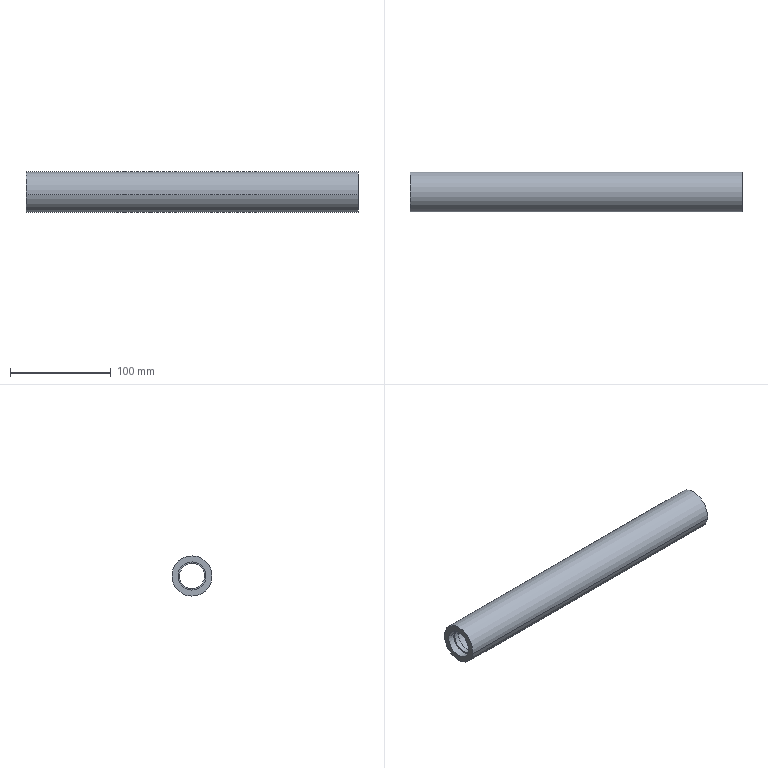Component | SolidWorks | 01-13MarkingMachinePrintingRoller-1 | 1 solid | 18 faces | box 330 x 40 x 40 mm | volume 123337 mm3 | cylinder 12 | plane 6 | commonest cylinder face diameters 28 x4 25 x4 40 x2 34 x2 | material A3 Steel
build123d program:
from build123d import *


with BuildPart() as part:
    # Sketch1 → Revolve1 (revolve)
    with BuildSketch(Plane.XY, mode=Mode.PRIVATE) as revolve1_sk:
        Polygon((-165, 20), (165, 20), (165, 14), (158, 14), (158, 12.5), (153, 12.5), (153, 17), (-153, 17), (-153, 12.5), (-158, 12.5), (-158, 14), (-165, 14), align=None)
    revolve(revolve1_sk.sketch.rotate(Axis((-220.554, 0, 0), (1, 0, 0)), 90), axis=Axis((-220.554, 0, 0), (1, 0, 0)))


solid = part.part

# Placed as in the assembly
solid = solid.moved(Location((-256.91, 2.41, 6.568), (0, 0, 0)))
STEP:
#1=COLOUR_RGB('',0.7922,0.8196,0.9333);
#2=FILL_AREA_STYLE_COLOUR('',#1);
#3=FILL_AREA_STYLE('',(#2));
#4=SURFACE_STYLE_FILL_AREA(#3);
#5=SURFACE_SIDE_STYLE('',(#4));
#6=SURFACE_STYLE_USAGE(.BOTH.,#5);
#7=PRESENTATION_STYLE_ASSIGNMENT((#6));
#8=CARTESIAN_POINT('',(-3.619,0.8756,0.3613));
#9=VERTEX_POINT('',#8);
#10=CARTESIAN_POINT('',(-3.619,-0.6858,0.1558));
#11=VERTEX_POINT('',#10);
#12=CARTESIAN_POINT('',(-3.619,0.0949,0.2586));
#13=DIRECTION('',(-1.,0.,0.));
#14=DIRECTION('',(0.,0.9915,0.1305));
#15=AXIS2_PLACEMENT_3D('',#12,#13,#14);
#16=CIRCLE('',#15,0.7874);
#17=EDGE_CURVE('',#9,#11,#16,.T.);
#18=ORIENTED_EDGE('',*,*,#17,.T.);
#19=CARTESIAN_POINT('',(-16.611,-0.6858,0.1558));
#20=VERTEX_POINT('',#19);
#21=CARTESIAN_POINT('',(-18.798,-0.6858,0.1558));
#22=DIRECTION('',(-1.,0.,0.));
#23=VECTOR('',#22,39.37);
#24=LINE('',#21,#23);
#25=EDGE_CURVE('',#11,#20,#24,.T.);
#26=ORIENTED_EDGE('',*,*,#25,.T.);
#27=CARTESIAN_POINT('',(-16.611,0.8756,0.3613));
#28=VERTEX_POINT('',#27);
#29=CARTESIAN_POINT('',(-16.611,0.0949,0.2586));
#30=DIRECTION('',(-1.,0.,0.));
#31=DIRECTION('',(0.,0.9915,0.1305));
#32=AXIS2_PLACEMENT_3D('',#29,#30,#31);
#33=CIRCLE('',#32,0.7874);
#34=EDGE_CURVE('',#28,#20,#33,.T.);
#35=ORIENTED_EDGE('',*,*,#34,.F.);
#36=CARTESIAN_POINT('',(-18.798,0.8756,0.3613));
#37=DIRECTION('',(-1.,0.,0.));
#38=VECTOR('',#37,39.37);
#39=LINE('',#36,#38);
#40=EDGE_CURVE('',#9,#28,#39,.T.);
#41=ORIENTED_EDGE('',*,*,#40,.F.);
#42=EDGE_LOOP('',(#18,#26,#35,#41));
#43=FACE_OUTER_BOUND('',#42,.T.);
#44=CARTESIAN_POINT('',(-18.798,0.0949,0.2586));
#45=DIRECTION('',(-1.,0.,0.));
#46=DIRECTION('',(0.,0.9915,0.1305));
#47=AXIS2_PLACEMENT_3D('',#44,#45,#46);
#48=CYLINDRICAL_SURFACE('',#47,0.7874);
#49=ADVANCED_FACE('',(#43),#48,.T.);
#50=CARTESIAN_POINT('',(-3.619,-0.4516,0.1867));
#51=VERTEX_POINT('',#50);
#52=CARTESIAN_POINT('',(-3.619,0.6414,0.3305));
#53=VERTEX_POINT('',#52);
#54=CARTESIAN_POINT('',(-3.619,0.0949,0.2586));
#55=DIRECTION('',(-1.,0.,0.));
#56=DIRECTION('',(0.,0.9915,0.1305));
#57=AXIS2_PLACEMENT_3D('',#54,#55,#56);
#58=CIRCLE('',#57,0.5512);
#59=EDGE_CURVE('',#51,#53,#58,.T.);
#60=ORIENTED_EDGE('',*,*,#59,.F.);
#61=CARTESIAN_POINT('',(-3.894,-0.4516,0.1867));
#62=VERTEX_POINT('',#61);
#63=CARTESIAN_POINT('',(-18.798,-0.4516,0.1867));
#64=DIRECTION('',(-1.,0.,0.));
#65=VECTOR('',#64,39.37);
#66=LINE('',#63,#65);
#67=EDGE_CURVE('',#51,#62,#66,.T.);
#68=ORIENTED_EDGE('',*,*,#67,.T.);
#69=CARTESIAN_POINT('',(-3.894,0.6414,0.3305));
#70=VERTEX_POINT('',#69);
#71=CARTESIAN_POINT('',(-3.894,0.0949,0.2586));
#72=DIRECTION('',(-1.,0.,0.));
#73=DIRECTION('',(0.,0.9915,0.1305));
#74=AXIS2_PLACEMENT_3D('',#71,#72,#73);
#75=CIRCLE('',#74,0.5512);
#76=EDGE_CURVE('',#62,#70,#75,.T.);
#77=ORIENTED_EDGE('',*,*,#76,.T.);
#78=CARTESIAN_POINT('',(-18.798,0.6414,0.3305));
#79=DIRECTION('',(-1.,0.,0.));
#80=VECTOR('',#79,39.37);
#81=LINE('',#78,#80);
#82=EDGE_CURVE('',#53,#70,#81,.T.);
#83=ORIENTED_EDGE('',*,*,#82,.F.);
#84=EDGE_LOOP('',(#60,#68,#77,#83));
#85=FACE_OUTER_BOUND('',#84,.T.);
#86=CARTESIAN_POINT('',(-18.798,0.0949,0.2586));
#87=DIRECTION('',(-1.,0.,0.));
#88=DIRECTION('',(0.,0.9915,0.1305));
#89=AXIS2_PLACEMENT_3D('',#86,#87,#88);
#90=CYLINDRICAL_SURFACE('',#89,0.5512);
#91=ADVANCED_FACE('',(#85),#90,.F.);
#92=CARTESIAN_POINT('',(-3.894,-0.393,0.1944));
#93=VERTEX_POINT('',#92);
#94=CARTESIAN_POINT('',(-3.894,0.5828,0.3228));
#95=VERTEX_POINT('',#94);
#96=CARTESIAN_POINT('',(-3.894,0.0949,0.2586));
#97=DIRECTION('',(-1.,0.,0.));
#98=DIRECTION('',(0.,0.9915,0.1305));
#99=AXIS2_PLACEMENT_3D('',#96,#97,#98);
#100=CIRCLE('',#99,0.4921);
#101=EDGE_CURVE('',#93,#95,#100,.T.);
#102=ORIENTED_EDGE('',*,*,#101,.F.);
#103=CARTESIAN_POINT('',(-4.091,-0.393,0.1944));
#104=VERTEX_POINT('',#103);
#105=CARTESIAN_POINT('',(-18.798,-0.393,0.1944));
#106=DIRECTION('',(-1.,0.,0.));
#107=VECTOR('',#106,39.37);
#108=LINE('',#105,#107);
#109=EDGE_CURVE('',#93,#104,#108,.T.);
#110=ORIENTED_EDGE('',*,*,#109,.T.);
#111=CARTESIAN_POINT('',(-4.091,0.5828,0.3228));
#112=VERTEX_POINT('',#111);
#113=CARTESIAN_POINT('',(-4.091,0.0949,0.2586));
#114=DIRECTION('',(-1.,0.,0.));
#115=DIRECTION('',(0.,0.9915,0.1305));
#116=AXIS2_PLACEMENT_3D('',#113,#114,#115);
#117=CIRCLE('',#116,0.4921);
#118=EDGE_CURVE('',#104,#112,#117,.T.);
#119=ORIENTED_EDGE('',*,*,#118,.T.);
#120=CARTESIAN_POINT('',(-18.798,0.5828,0.3228));
#121=DIRECTION('',(-1.,0.,0.));
#122=VECTOR('',#121,39.37);
#123=LINE('',#120,#122);
#124=EDGE_CURVE('',#95,#112,#123,.T.);
#125=ORIENTED_EDGE('',*,*,#124,.F.);
#126=EDGE_LOOP('',(#102,#110,#119,#125));
#127=FACE_OUTER_BOUND('',#126,.T.);
#128=CARTESIAN_POINT('',(-18.798,0.0949,0.2586));
#129=DIRECTION('',(-1.,0.,0.));
#130=DIRECTION('',(0.,0.9915,0.1305));
#131=AXIS2_PLACEMENT_3D('',#128,#129,#130);
#132=CYLINDRICAL_SURFACE('',#131,0.4921);
#133=ADVANCED_FACE('',(#127),#132,.F.);
#134=CARTESIAN_POINT('',(-4.091,-0.5687,0.1713));
#135=VERTEX_POINT('',#134);
#136=CARTESIAN_POINT('',(-4.091,0.7585,0.3459));
#137=VERTEX_POINT('',#136);
#138=CARTESIAN_POINT('',(-4.091,0.0949,0.2586));
#139=DIRECTION('',(-1.,0.,0.));
#140=DIRECTION('',(0.,0.9915,0.1305));
#141=AXIS2_PLACEMENT_3D('',#138,#139,#140);
#142=CIRCLE('',#141,0.6693);
#143=EDGE_CURVE('',#135,#137,#142,.T.);
#144=ORIENTED_EDGE('',*,*,#143,.F.);
#145=CARTESIAN_POINT('',(-16.138,-0.5687,0.1713));
#146=VERTEX_POINT('',#145);
#147=CARTESIAN_POINT('',(-18.798,-0.5687,0.1713));
#148=DIRECTION('',(-1.,0.,0.));
#149=VECTOR('',#148,39.37);
#150=LINE('',#147,#149);
#151=EDGE_CURVE('',#135,#146,#150,.T.);
#152=ORIENTED_EDGE('',*,*,#151,.T.);
#153=CARTESIAN_POINT('',(-16.138,0.7585,0.3459));
#154=VERTEX_POINT('',#153);
#155=CARTESIAN_POINT('',(-16.138,0.0949,0.2586));
#156=DIRECTION('',(-1.,0.,0.));
#157=DIRECTION('',(0.,0.9915,0.1305));
#158=AXIS2_PLACEMENT_3D('',#155,#156,#157);
#159=CIRCLE('',#158,0.6693);
#160=EDGE_CURVE('',#146,#154,#159,.T.);
#161=ORIENTED_EDGE('',*,*,#160,.T.);
#162=CARTESIAN_POINT('',(-18.798,0.7585,0.3459));
#163=DIRECTION('',(-1.,0.,0.));
#164=VECTOR('',#163,39.37);
#165=LINE('',#162,#164);
#166=EDGE_CURVE('',#137,#154,#165,.T.);
#167=ORIENTED_EDGE('',*,*,#166,.F.);
#168=EDGE_LOOP('',(#144,#152,#161,#167));
#169=FACE_OUTER_BOUND('',#168,.T.);
#170=CARTESIAN_POINT('',(-18.798,0.0949,0.2586));
#171=DIRECTION('',(-1.,0.,0.));
#172=DIRECTION('',(0.,0.9915,0.1305));
#173=AXIS2_PLACEMENT_3D('',#170,#171,#172);
#174=CYLINDRICAL_SURFACE('',#173,0.6693);
#175=ADVANCED_FACE('',(#169),#174,.F.);
#176=CARTESIAN_POINT('',(-16.138,-0.393,0.1944));
#177=VERTEX_POINT('',#176);
#178=CARTESIAN_POINT('',(-16.138,0.5828,0.3228));
#179=VERTEX_POINT('',#178);
#180=CARTESIAN_POINT('',(-16.138,0.0949,0.2586));
#181=DIRECTION('',(-1.,0.,0.));
#182=DIRECTION('',(0.,0.9915,0.1305));
#183=AXIS2_PLACEMENT_3D('',#180,#181,#182);
#184=CIRCLE('',#183,0.4921);
#185=EDGE_CURVE('',#177,#179,#184,.T.);
#186=ORIENTED_EDGE('',*,*,#185,.F.);
#187=CARTESIAN_POINT('',(-16.335,-0.393,0.1944));
#188=VERTEX_POINT('',#187);
#189=CARTESIAN_POINT('',(-18.798,-0.393,0.1944));
#190=DIRECTION('',(-1.,0.,0.));
#191=VECTOR('',#190,39.37);
#192=LINE('',#189,#191);
#193=EDGE_CURVE('',#177,#188,#192,.T.);
#194=ORIENTED_EDGE('',*,*,#193,.T.);
#195=CARTESIAN_POINT('',(-16.335,0.5828,0.3228));
#196=VERTEX_POINT('',#195);
#197=CARTESIAN_POINT('',(-16.335,0.0949,0.2586));
#198=DIRECTION('',(-1.,0.,0.));
#199=DIRECTION('',(0.,0.9915,0.1305));
#200=AXIS2_PLACEMENT_3D('',#197,#198,#199);
#201=CIRCLE('',#200,0.4921);
#202=EDGE_CURVE('',#188,#196,#201,.T.);
#203=ORIENTED_EDGE('',*,*,#202,.T.);
#204=CARTESIAN_POINT('',(-18.798,0.5828,0.3228));
#205=DIRECTION('',(-1.,0.,0.));
#206=VECTOR('',#205,39.37);
#207=LINE('',#204,#206);
#208=EDGE_CURVE('',#179,#196,#207,.T.);
#209=ORIENTED_EDGE('',*,*,#208,.F.);
#210=EDGE_LOOP('',(#186,#194,#203,#209));
#211=FACE_OUTER_BOUND('',#210,.T.);
#212=CARTESIAN_POINT('',(-18.798,0.0949,0.2586));
#213=DIRECTION('',(-1.,0.,0.));
#214=DIRECTION('',(0.,0.9915,0.1305));
#215=AXIS2_PLACEMENT_3D('',#212,#213,#214);
#216=CYLINDRICAL_SURFACE('',#215,0.4921);
#217=ADVANCED_FACE('',(#211),#216,.F.);
#218=CARTESIAN_POINT('',(-16.335,-0.4516,0.1867));
#219=VERTEX_POINT('',#218);
#220=CARTESIAN_POINT('',(-16.335,0.6414,0.3305));
#221=VERTEX_POINT('',#220);
#222=CARTESIAN_POINT('',(-16.335,0.0949,0.2586));
#223=DIRECTION('',(-1.,0.,0.));
#224=DIRECTION('',(0.,0.9915,0.1305));
#225=AXIS2_PLACEMENT_3D('',#222,#223,#224);
#226=CIRCLE('',#225,0.5512);
#227=EDGE_CURVE('',#219,#221,#226,.T.);
#228=ORIENTED_EDGE('',*,*,#227,.F.);
#229=CARTESIAN_POINT('',(-16.611,-0.4516,0.1867));
#230=VERTEX_POINT('',#229);
#231=CARTESIAN_POINT('',(-18.798,-0.4516,0.1867));
#232=DIRECTION('',(-1.,0.,0.));
#233=VECTOR('',#232,39.37);
#234=LINE('',#231,#233);
#235=EDGE_CURVE('',#219,#230,#234,.T.);
#236=ORIENTED_EDGE('',*,*,#235,.T.);
#237=CARTESIAN_POINT('',(-16.611,0.6414,0.3305));
#238=VERTEX_POINT('',#237);
#239=CARTESIAN_POINT('',(-16.611,0.0949,0.2586));
#240=DIRECTION('',(-1.,0.,0.));
#241=DIRECTION('',(0.,0.9915,0.1305));
#242=AXIS2_PLACEMENT_3D('',#239,#240,#241);
#243=CIRCLE('',#242,0.5512);
#244=EDGE_CURVE('',#230,#238,#243,.T.);
#245=ORIENTED_EDGE('',*,*,#244,.T.);
#246=CARTESIAN_POINT('',(-18.798,0.6414,0.3305));
#247=DIRECTION('',(-1.,0.,0.));
#248=VECTOR('',#247,39.37);
#249=LINE('',#246,#248);
#250=EDGE_CURVE('',#221,#238,#249,.T.);
#251=ORIENTED_EDGE('',*,*,#250,.F.);
#252=EDGE_LOOP('',(#228,#236,#245,#251));
#253=FACE_OUTER_BOUND('',#252,.T.);
#254=CARTESIAN_POINT('',(-18.798,0.0949,0.2586));
#255=DIRECTION('',(-1.,0.,0.));
#256=DIRECTION('',(0.,0.9915,0.1305));
#257=AXIS2_PLACEMENT_3D('',#254,#255,#256);
#258=CYLINDRICAL_SURFACE('',#257,0.5512);
#259=ADVANCED_FACE('',(#253),#258,.F.);
#260=CARTESIAN_POINT('',(-16.611,0.0949,0.2586));
#261=DIRECTION('',(-1.,0.,0.));
#262=DIRECTION('',(0.,0.9915,0.1305));
#263=AXIS2_PLACEMENT_3D('',#260,#261,#262);
#264=CIRCLE('',#263,0.5512);
#265=EDGE_CURVE('',#238,#230,#264,.T.);
#266=ORIENTED_EDGE('',*,*,#265,.F.);
#267=ORIENTED_EDGE('',*,*,#244,.F.);
#268=EDGE_LOOP('',(#266,#267));
#269=FACE_BOUND('',#268,.T.);
#270=ORIENTED_EDGE('',*,*,#34,.T.);
#271=CARTESIAN_POINT('',(-16.611,0.0949,0.2586));
#272=DIRECTION('',(-1.,0.,0.));
#273=DIRECTION('',(0.,0.9915,0.1305));
#274=AXIS2_PLACEMENT_3D('',#271,#272,#273);
#275=CIRCLE('',#274,0.7874);
#276=EDGE_CURVE('',#20,#28,#275,.T.);
#277=ORIENTED_EDGE('',*,*,#276,.T.);
#278=EDGE_LOOP('',(#270,#277));
#279=FACE_OUTER_BOUND('',#278,.T.);
#280=CARTESIAN_POINT('',(-16.611,0.1976,-0.5221));
#281=DIRECTION('',(1.,0.,0.));
#282=DIRECTION('',(0.,-0.9915,-0.1305));
#283=AXIS2_PLACEMENT_3D('',#280,#281,#282);
#284=PLANE('',#283);
#285=ADVANCED_FACE('',(#269,#279),#284,.F.);
#286=ORIENTED_EDGE('',*,*,#235,.F.);
#287=CARTESIAN_POINT('',(-16.335,0.0949,0.2586));
#288=DIRECTION('',(-1.,0.,0.));
#289=DIRECTION('',(0.,0.9915,0.1305));
#290=AXIS2_PLACEMENT_3D('',#287,#288,#289);
#291=CIRCLE('',#290,0.5512);
#292=EDGE_CURVE('',#221,#219,#291,.T.);
#293=ORIENTED_EDGE('',*,*,#292,.F.);
#294=ORIENTED_EDGE('',*,*,#250,.T.);
#295=ORIENTED_EDGE('',*,*,#265,.T.);
#296=EDGE_LOOP('',(#286,#293,#294,#295));
#297=FACE_OUTER_BOUND('',#296,.T.);
#298=CARTESIAN_POINT('',(-18.798,0.0949,0.2586));
#299=DIRECTION('',(-1.,0.,0.));
#300=DIRECTION('',(0.,0.9915,0.1305));
#301=AXIS2_PLACEMENT_3D('',#298,#299,#300);
#302=CYLINDRICAL_SURFACE('',#301,0.5512);
#303=ADVANCED_FACE('',(#297),#302,.F.);
#304=CARTESIAN_POINT('',(-16.335,0.0949,0.2586));
#305=DIRECTION('',(-1.,0.,0.));
#306=DIRECTION('',(0.,0.9915,0.1305));
#307=AXIS2_PLACEMENT_3D('',#304,#305,#306);
#308=CIRCLE('',#307,0.4921);
#309=EDGE_CURVE('',#196,#188,#308,.T.);
#310=ORIENTED_EDGE('',*,*,#309,.F.);
#311=ORIENTED_EDGE('',*,*,#202,.F.);
#312=EDGE_LOOP('',(#310,#311));
#313=FACE_BOUND('',#312,.T.);
#314=ORIENTED_EDGE('',*,*,#292,.T.);
#315=ORIENTED_EDGE('',*,*,#227,.T.);
#316=EDGE_LOOP('',(#314,#315));
#317=FACE_OUTER_BOUND('',#316,.T.);
#318=CARTESIAN_POINT('',(-16.335,0.1668,-0.2879));
#319=DIRECTION('',(1.,0.,0.));
#320=DIRECTION('',(0.,-0.9915,-0.1305));
#321=AXIS2_PLACEMENT_3D('',#318,#319,#320);
#322=PLANE('',#321);
#323=ADVANCED_FACE('',(#313,#317),#322,.F.);
#324=ORIENTED_EDGE('',*,*,#193,.F.);
#325=CARTESIAN_POINT('',(-16.138,0.0949,0.2586));
#326=DIRECTION('',(-1.,0.,0.));
#327=DIRECTION('',(0.,0.9915,0.1305));
#328=AXIS2_PLACEMENT_3D('',#325,#326,#327);
#329=CIRCLE('',#328,0.4921);
#330=EDGE_CURVE('',#179,#177,#329,.T.);
#331=ORIENTED_EDGE('',*,*,#330,.F.);
#332=ORIENTED_EDGE('',*,*,#208,.T.);
#333=ORIENTED_EDGE('',*,*,#309,.T.);
#334=EDGE_LOOP('',(#324,#331,#332,#333));
#335=FACE_OUTER_BOUND('',#334,.T.);
#336=CARTESIAN_POINT('',(-18.798,0.0949,0.2586));
#337=DIRECTION('',(-1.,0.,0.));
#338=DIRECTION('',(0.,0.9915,0.1305));
#339=AXIS2_PLACEMENT_3D('',#336,#337,#338);
#340=CYLINDRICAL_SURFACE('',#339,0.4921);
#341=ADVANCED_FACE('',(#335),#340,.F.);
#342=CARTESIAN_POINT('',(-16.138,0.0949,0.2586));
#343=DIRECTION('',(-1.,0.,0.));
#344=DIRECTION('',(0.,0.9915,0.1305));
#345=AXIS2_PLACEMENT_3D('',#342,#343,#344);
#346=CIRCLE('',#345,0.6693);
#347=EDGE_CURVE('',#154,#146,#346,.T.);
#348=ORIENTED_EDGE('',*,*,#347,.F.);
#349=ORIENTED_EDGE('',*,*,#160,.F.);
#350=EDGE_LOOP('',(#348,#349));
#351=FACE_OUTER_BOUND('',#350,.T.);
#352=ORIENTED_EDGE('',*,*,#330,.T.);
#353=ORIENTED_EDGE('',*,*,#185,.T.);
#354=EDGE_LOOP('',(#352,#353));
#355=FACE_BOUND('',#354,.T.);
#356=CARTESIAN_POINT('',(-16.138,0.1591,-0.2293));
#357=DIRECTION('',(-1.,0.,0.));
#358=DIRECTION('',(0.,0.9915,0.1305));
#359=AXIS2_PLACEMENT_3D('',#356,#357,#358);
#360=PLANE('',#359);
#361=ADVANCED_FACE('',(#351,#355),#360,.F.);
#362=ORIENTED_EDGE('',*,*,#151,.F.);
#363=CARTESIAN_POINT('',(-4.091,0.0949,0.2586));
#364=DIRECTION('',(-1.,0.,0.));
#365=DIRECTION('',(0.,0.9915,0.1305));
#366=AXIS2_PLACEMENT_3D('',#363,#364,#365);
#367=CIRCLE('',#366,0.6693);
#368=EDGE_CURVE('',#137,#135,#367,.T.);
#369=ORIENTED_EDGE('',*,*,#368,.F.);
#370=ORIENTED_EDGE('',*,*,#166,.T.);
#371=ORIENTED_EDGE('',*,*,#347,.T.);
#372=EDGE_LOOP('',(#362,#369,#370,#371));
#373=FACE_OUTER_BOUND('',#372,.T.);
#374=CARTESIAN_POINT('',(-18.798,0.0949,0.2586));
#375=DIRECTION('',(-1.,0.,0.));
#376=DIRECTION('',(0.,0.9915,0.1305));
#377=AXIS2_PLACEMENT_3D('',#374,#375,#376);
#378=CYLINDRICAL_SURFACE('',#377,0.6693);
#379=ADVANCED_FACE('',(#373),#378,.F.);
#380=CARTESIAN_POINT('',(-4.091,0.0949,0.2586));
#381=DIRECTION('',(-1.,0.,0.));
#382=DIRECTION('',(0.,0.9915,0.1305));
#383=AXIS2_PLACEMENT_3D('',#380,#381,#382);
#384=CIRCLE('',#383,0.4921);
#385=EDGE_CURVE('',#112,#104,#384,.T.);
#386=ORIENTED_EDGE('',*,*,#385,.F.);
#387=ORIENTED_EDGE('',*,*,#118,.F.);
#388=EDGE_LOOP('',(#386,#387));
#389=FACE_BOUND('',#388,.T.);
#390=ORIENTED_EDGE('',*,*,#368,.T.);
#391=ORIENTED_EDGE('',*,*,#143,.T.);
#392=EDGE_LOOP('',(#390,#391));
#393=FACE_OUTER_BOUND('',#392,.T.);
#394=CARTESIAN_POINT('',(-4.091,0.1591,-0.2293));
#395=DIRECTION('',(1.,0.,0.));
#396=DIRECTION('',(0.,-0.9915,-0.1305));
#397=AXIS2_PLACEMENT_3D('',#394,#395,#396);
#398=PLANE('',#397);
#399=ADVANCED_FACE('',(#389,#393),#398,.F.);
#400=ORIENTED_EDGE('',*,*,#109,.F.);
#401=CARTESIAN_POINT('',(-3.894,0.0949,0.2586));
#402=DIRECTION('',(-1.,0.,0.));
#403=DIRECTION('',(0.,0.9915,0.1305));
#404=AXIS2_PLACEMENT_3D('',#401,#402,#403);
#405=CIRCLE('',#404,0.4921);
#406=EDGE_CURVE('',#95,#93,#405,.T.);
#407=ORIENTED_EDGE('',*,*,#406,.F.);
#408=ORIENTED_EDGE('',*,*,#124,.T.);
#409=ORIENTED_EDGE('',*,*,#385,.T.);
#410=EDGE_LOOP('',(#400,#407,#408,#409));
#411=FACE_OUTER_BOUND('',#410,.T.);
#412=CARTESIAN_POINT('',(-18.798,0.0949,0.2586));
#413=DIRECTION('',(-1.,0.,0.));
#414=DIRECTION('',(0.,0.9915,0.1305));
#415=AXIS2_PLACEMENT_3D('',#412,#413,#414);
#416=CYLINDRICAL_SURFACE('',#415,0.4921);
#417=ADVANCED_FACE('',(#411),#416,.F.);
#418=CARTESIAN_POINT('',(-3.894,0.0949,0.2586));
#419=DIRECTION('',(-1.,0.,0.));
#420=DIRECTION('',(0.,0.9915,0.1305));
#421=AXIS2_PLACEMENT_3D('',#418,#419,#420);
#422=CIRCLE('',#421,0.5512);
#423=EDGE_CURVE('',#70,#62,#422,.T.);
#424=ORIENTED_EDGE('',*,*,#423,.F.);
#425=ORIENTED_EDGE('',*,*,#76,.F.);
#426=EDGE_LOOP('',(#424,#425));
#427=FACE_OUTER_BOUND('',#426,.T.);
#428=ORIENTED_EDGE('',*,*,#406,.T.);
#429=ORIENTED_EDGE('',*,*,#101,.T.);
#430=EDGE_LOOP('',(#428,#429));
#431=FACE_BOUND('',#430,.T.);
#432=CARTESIAN_POINT('',(-3.894,0.1668,-0.2879));
#433=DIRECTION('',(-1.,0.,0.));
#434=DIRECTION('',(0.,0.9915,0.1305));
#435=AXIS2_PLACEMENT_3D('',#432,#433,#434);
#436=PLANE('',#435);
#437=ADVANCED_FACE('',(#427,#431),#436,.F.);
#438=ORIENTED_EDGE('',*,*,#67,.F.);
#439=CARTESIAN_POINT('',(-3.619,0.0949,0.2586));
#440=DIRECTION('',(-1.,0.,0.));
#441=DIRECTION('',(0.,0.9915,0.1305));
#442=AXIS2_PLACEMENT_3D('',#439,#440,#441);
#443=CIRCLE('',#442,0.5512);
#444=EDGE_CURVE('',#53,#51,#443,.T.);
#445=ORIENTED_EDGE('',*,*,#444,.F.);
#446=ORIENTED_EDGE('',*,*,#82,.T.);
#447=ORIENTED_EDGE('',*,*,#423,.T.);
#448=EDGE_LOOP('',(#438,#445,#446,#447));
#449=FACE_OUTER_BOUND('',#448,.T.);
#450=CARTESIAN_POINT('',(-18.798,0.0949,0.2586));
#451=DIRECTION('',(-1.,0.,0.));
#452=DIRECTION('',(0.,0.9915,0.1305));
#453=AXIS2_PLACEMENT_3D('',#450,#451,#452);
#454=CYLINDRICAL_SURFACE('',#453,0.5512);
#455=ADVANCED_FACE('',(#449),#454,.F.);
#456=ORIENTED_EDGE('',*,*,#17,.F.);
#457=CARTESIAN_POINT('',(-3.619,0.0949,0.2586));
#458=DIRECTION('',(-1.,0.,0.));
#459=DIRECTION('',(0.,0.9915,0.1305));
#460=AXIS2_PLACEMENT_3D('',#457,#458,#459);
#461=CIRCLE('',#460,0.7874);
#462=EDGE_CURVE('',#11,#9,#461,.T.);
#463=ORIENTED_EDGE('',*,*,#462,.F.);
#464=EDGE_LOOP('',(#456,#463));
#465=FACE_OUTER_BOUND('',#464,.T.);
#466=ORIENTED_EDGE('',*,*,#444,.T.);
#467=ORIENTED_EDGE('',*,*,#59,.T.);
#468=EDGE_LOOP('',(#466,#467));
#469=FACE_BOUND('',#468,.T.);
#470=CARTESIAN_POINT('',(-3.619,0.1976,-0.5221));
#471=DIRECTION('',(-1.,0.,0.));
#472=DIRECTION('',(0.,0.9915,0.1305));
#473=AXIS2_PLACEMENT_3D('',#470,#471,#472);
#474=PLANE('',#473);
#475=ADVANCED_FACE('',(#465,#469),#474,.F.);
#476=ORIENTED_EDGE('',*,*,#25,.F.);
#477=ORIENTED_EDGE('',*,*,#462,.T.);
#478=ORIENTED_EDGE('',*,*,#40,.T.);
#479=ORIENTED_EDGE('',*,*,#276,.F.);
#480=EDGE_LOOP('',(#476,#477,#478,#479));
#481=FACE_OUTER_BOUND('',#480,.T.);
#482=CARTESIAN_POINT('',(-18.798,0.0949,0.2586));
#483=DIRECTION('',(-1.,0.,0.));
#484=DIRECTION('',(0.,0.9915,0.1305));
#485=AXIS2_PLACEMENT_3D('',#482,#483,#484);
#486=CYLINDRICAL_SURFACE('',#485,0.7874);
#487=ADVANCED_FACE('',(#481),#486,.T.);
#488=CLOSED_SHELL('',(#49,#91,#133,#175,#217,#259,#285,#303,#323,#341,#361,#379,#399,#417,#437,#455,#475,#487));
#489=MANIFOLD_SOLID_BREP('',#488);
#490=STYLED_ITEM('',(#7),#489);
#491=PRESENTATION_LAYER_ASSIGNMENT('','',(#490));
#492=(LENGTH_UNIT()NAMED_UNIT(*)SI_UNIT($,.METRE.));
#493=LENGTH_MEASURE_WITH_UNIT(LENGTH_MEASURE(0.0254),#492);
#494=DIMENSIONAL_EXPONENTS(1.,0.,0.,0.,0.,0.,0.);
#495=(CONVERSION_BASED_UNIT('',#493)LENGTH_UNIT()NAMED_UNIT(#494));
#496=UNCERTAINTY_MEASURE_WITH_UNIT(LENGTH_MEASURE(0.00001),#495,'','');
#497=(NAMED_UNIT(*)PLANE_ANGLE_UNIT()SI_UNIT($,.RADIAN.));
#498=(NAMED_UNIT(*)SI_UNIT($,.STERADIAN.)SOLID_ANGLE_UNIT());
#499=(GEOMETRIC_REPRESENTATION_CONTEXT(3)GLOBAL_UNCERTAINTY_ASSIGNED_CONTEXT((#496))GLOBAL_UNIT_ASSIGNED_CONTEXT((#495,#497,#498))REPRESENTATION_CONTEXT('',''));
#500=MECHANICAL_DESIGN_GEOMETRIC_PRESENTATION_REPRESENTATION('',(#490),#499);
#501=CARTESIAN_POINT('',(0.,0.,0.));
#502=DIRECTION('',(0.,0.,1.));
#503=DIRECTION('',(1.,0.,0.));
#504=AXIS2_PLACEMENT_3D('',#501,#502,#503);
#505=(LENGTH_UNIT()NAMED_UNIT(*)SI_UNIT($,.METRE.));
#506=LENGTH_MEASURE_WITH_UNIT(LENGTH_MEASURE(0.0254),#505);
#507=DIMENSIONAL_EXPONENTS(1.,0.,0.,0.,0.,0.,0.);
#508=(CONVERSION_BASED_UNIT('',#506)LENGTH_UNIT()NAMED_UNIT(#507));
#509=UNCERTAINTY_MEASURE_WITH_UNIT(LENGTH_MEASURE(0.00001),#508,'','');
#510=(NAMED_UNIT(*)PLANE_ANGLE_UNIT()SI_UNIT($,.RADIAN.));
#511=(NAMED_UNIT(*)SI_UNIT($,.STERADIAN.)SOLID_ANGLE_UNIT());
#512=(GEOMETRIC_REPRESENTATION_CONTEXT(3)GLOBAL_UNCERTAINTY_ASSIGNED_CONTEXT((#509))GLOBAL_UNIT_ASSIGNED_CONTEXT((#508,#510,#511))REPRESENTATION_CONTEXT('',''));
#513=ADVANCED_BREP_SHAPE_REPRESENTATION('',(#489,#504),#512);